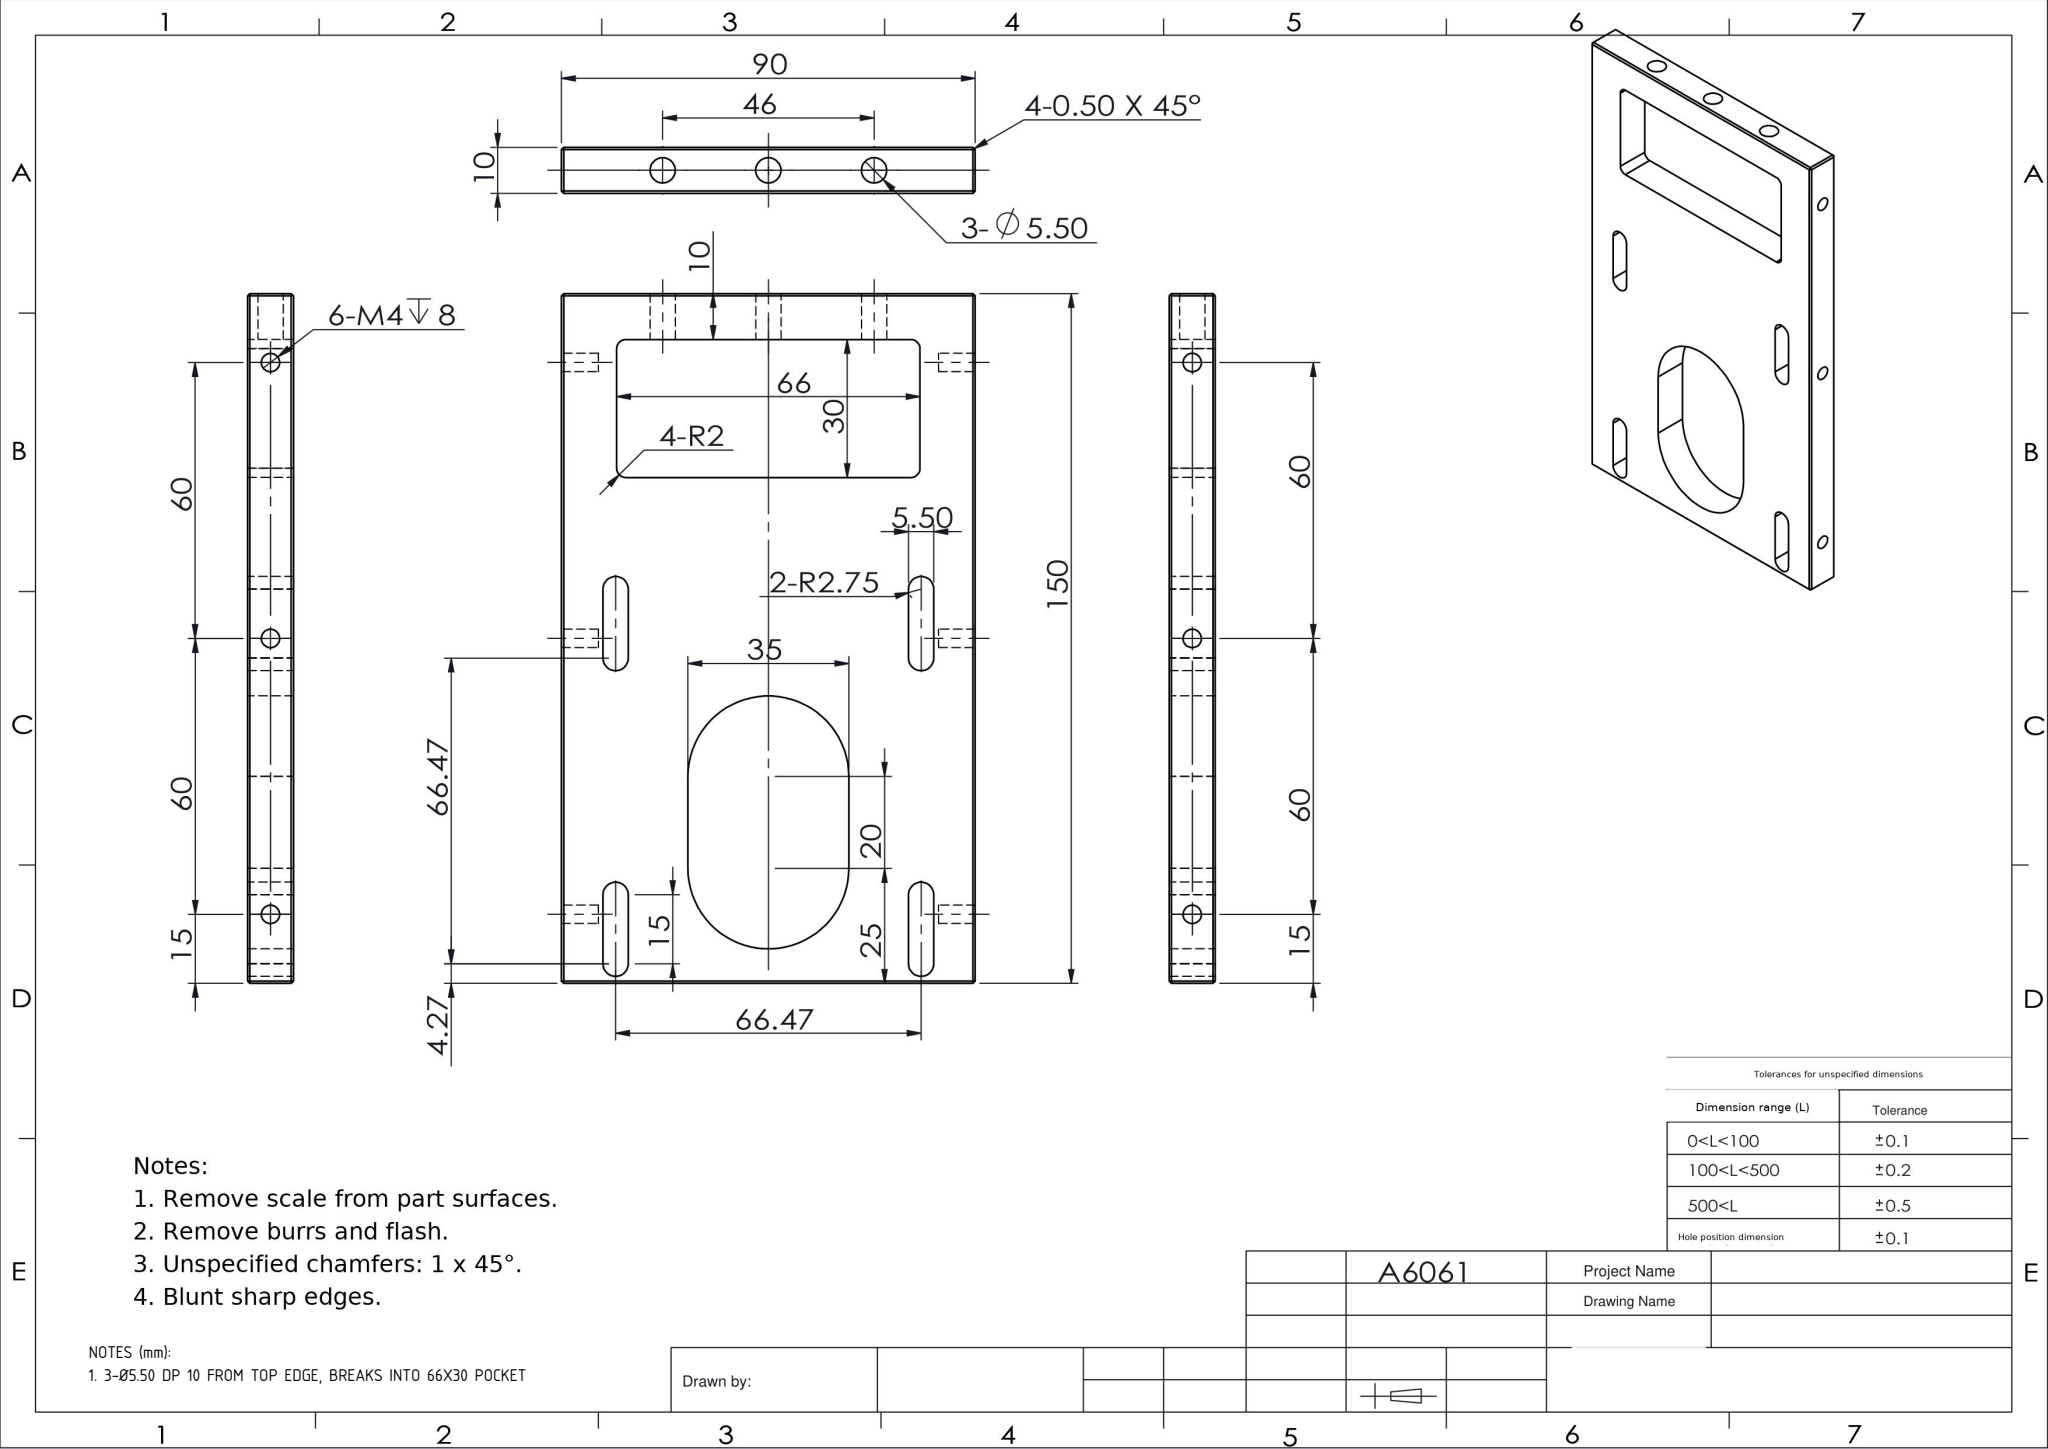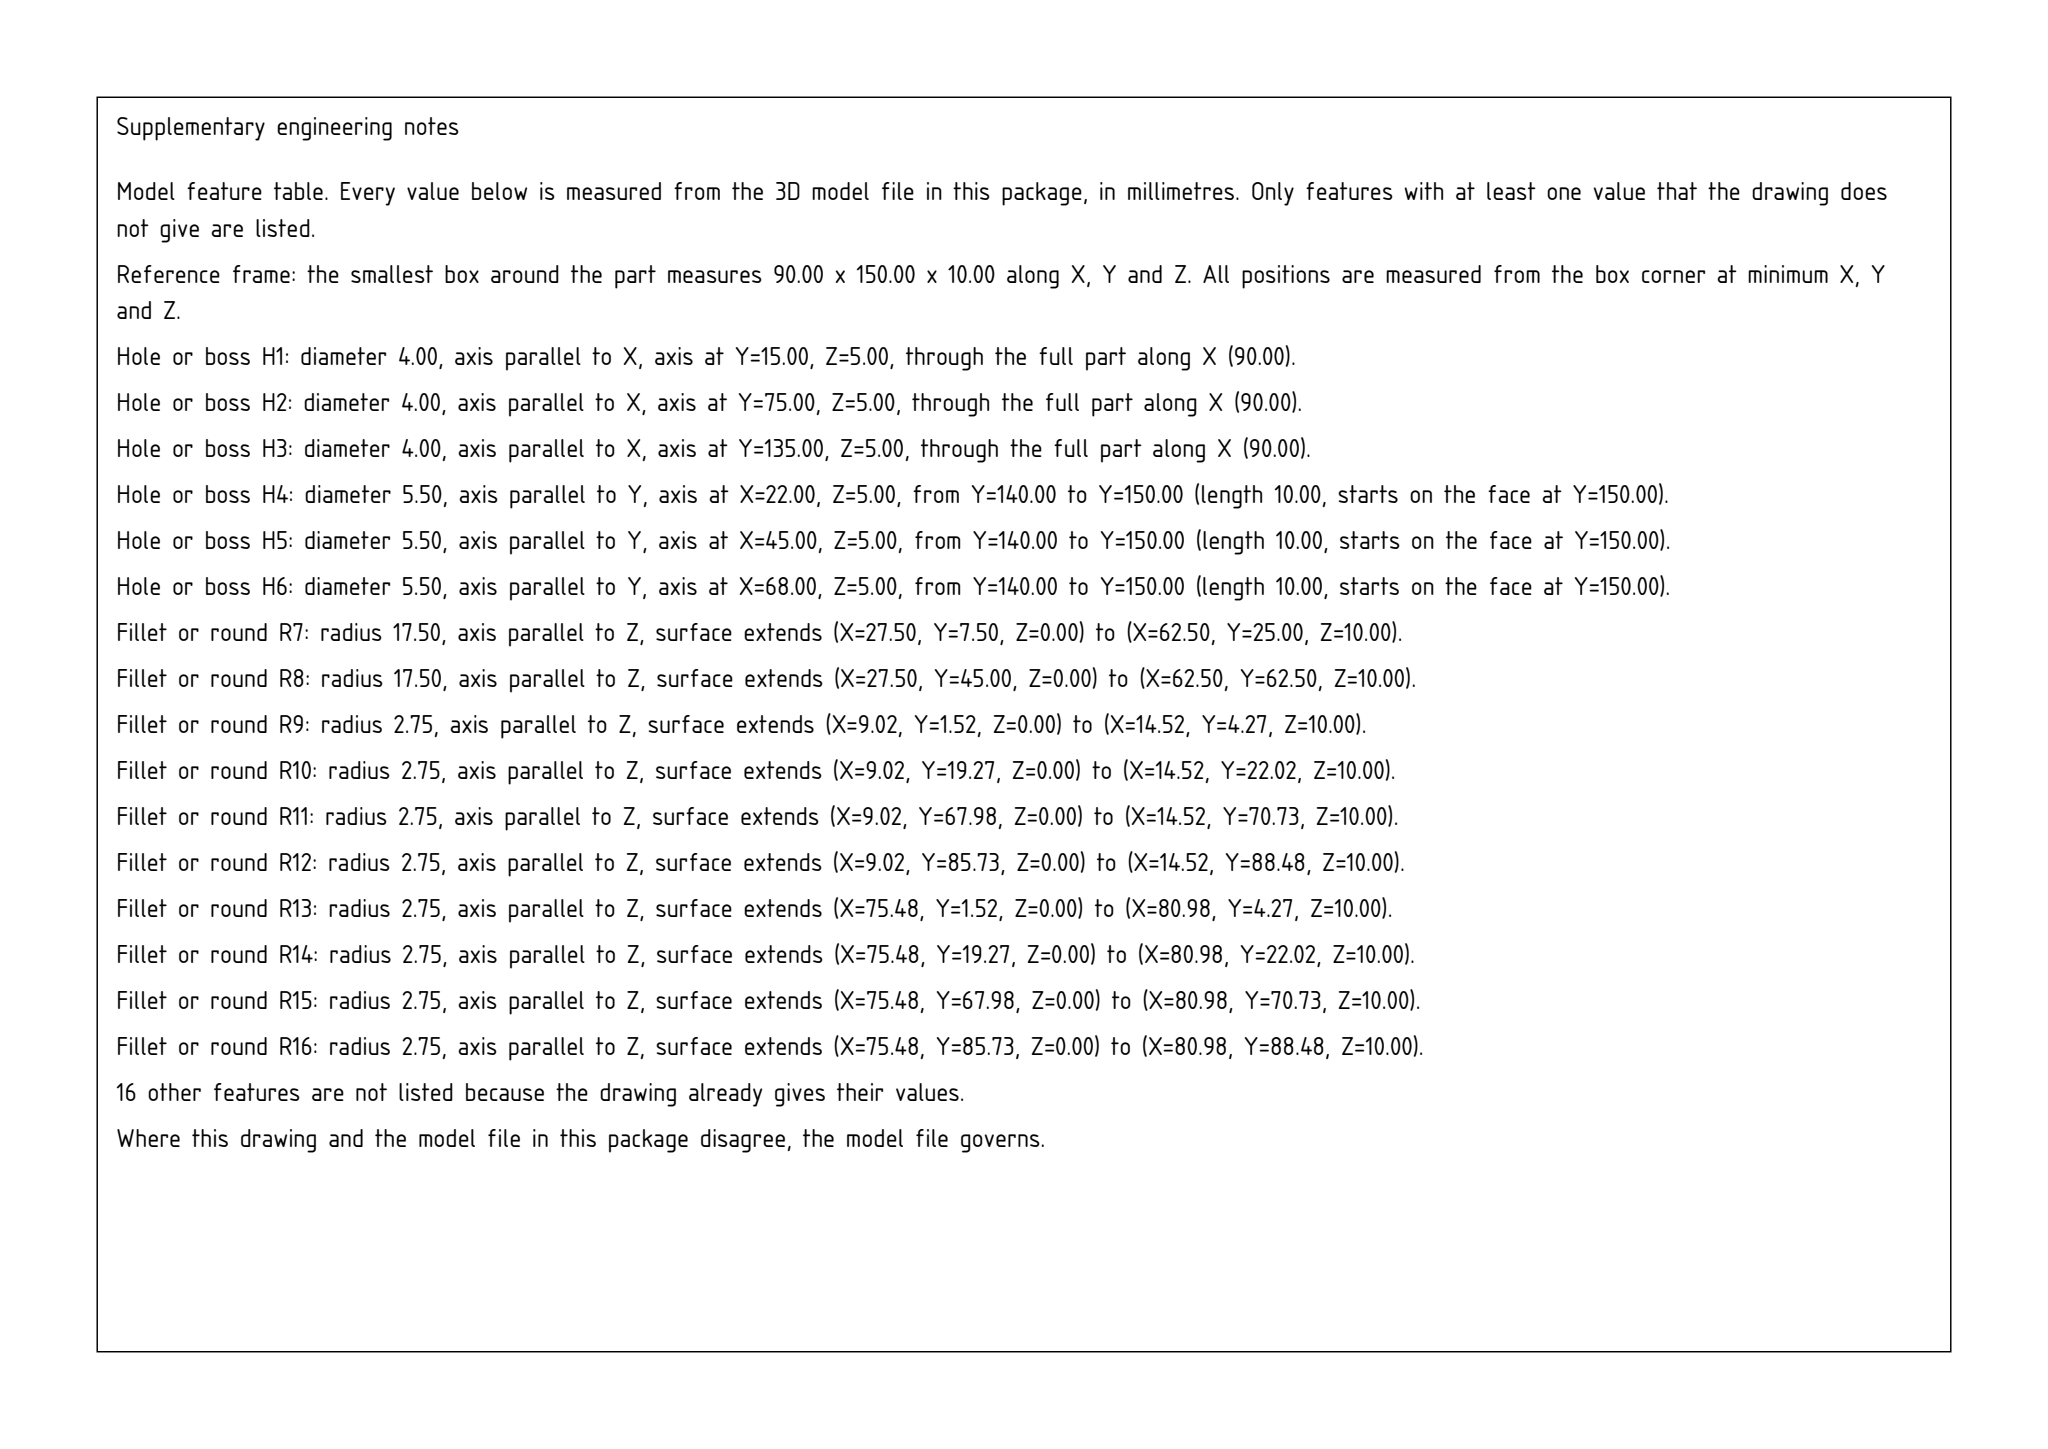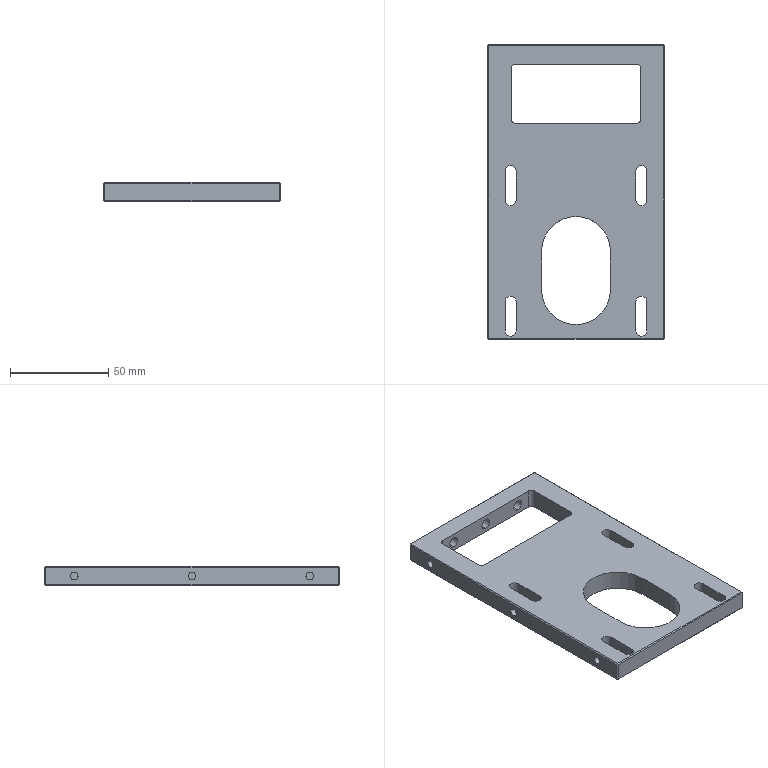Part | SolidWorks | mm | 1 solid | 78 faces | box 90 x 150 x 10 mm | volume 92923 mm3 | plane 46 | cylinder 32 | commonest cylinder face diameters 4 x16 5.5 x14 35 x2
Drawing notes:
3-Ø5.50 DP 10 FROM TOP EDGE, BREAKS INTO 66X30 POCKET | from the solid: Cyl dia5.5 axis y at x=22,45,68, z=5, len 10; from y=150 face to pocket face y=140
build123d program:
from build123d import *

# Parameters (mm, degrees)
SKETCH1_W           = 90
SKETCH1_H           = 150
BOSS_EXTRUDE1_DEPTH = 5
SKETCH5_R           = 2.1
CUT_EXTRUDE1_DEPTH  = 89.034
SKETCH6_R           = 17.5
CUT_EXTRUDE2_DEPTH  = 89.034
CHAMFER1_SIZE       = 0.5
CUT_EXTRUDE3_DEPTH  = 89.034
CUT_EXTRUDE4_DEPTH  = 89.034
SKETCH11_W          = 66
SKETCH11_H          = 30
CUT_EXTRUDE5_DEPTH  = 89.034
FILLET1_R           = 2
SKETCH13_R          = 2.75
CUT_EXTRUDE6_DEPTH  = 20
SKETCH14_R          = 2
CUT_EXTRUDE7_DEPTH  = 8
LPATTERN1_COUNT     = 3
LPATTERN1_PITCH     = 60
CUT_EXTRUDE8_START  = -8
SKETCH15_R          = 2
CUT_EXTRUDE8_DEPTH  = 8
LPATTERN2_COUNT     = 3
LPATTERN2_PITCH     = 60


with BuildPart() as part:
    # Sketch1 → Boss-Extrude1 (new, symmetric)
    with BuildSketch(Plane.XY):
        Rectangle(SKETCH1_W, SKETCH1_H)
    extrude(amount=BOSS_EXTRUDE1_DEPTH, both=True)

    # Sketch5 → Cut-Extrude1 (cut, through all)
    with BuildSketch(Plane(origin=(0, 0, -5), x_dir=(-1, 0, 0), z_dir=(0, 0, -1))):
        with Locations((-33.234, 3.234)):
            Circle(SKETCH5_R)
        with Locations((33.234, 3.234)):
            Circle(SKETCH5_R)
        with Locations((-33.234, -63.234)):
            Circle(SKETCH5_R)
        with Locations((33.234, -63.234)):
            Circle(SKETCH5_R)
    extrude(amount=-CUT_EXTRUDE1_DEPTH, mode=Mode.SUBTRACT)

    # Sketch6 → Cut-Extrude2 (cut, through all)
    with BuildSketch(Plane.XY.offset(5)):
        with Locations((0, -42)):
            Circle(SKETCH6_R)
    extrude(amount=-CUT_EXTRUDE2_DEPTH, mode=Mode.SUBTRACT)

    # Chamfer1
    chamfer1_edges = [part.edges().sort_by_distance(p)[0] for p in [
        (-45, 0, 5),
        (0, -75, 5),
        (45, 0, 5),
        (0, -75, -5),
        (-45, 0, -5),
        (0, 75, -5),
        (45, 0, -5),
        (0, 75, 5),
        (45, -75, 0),
        (-45, -75, 0),
        (-45, 75, 0),
        (45, 75, 0),
    ]]
    chamfer(chamfer1_edges, length=CHAMFER1_SIZE)

    # Sketch9 → Cut-Extrude3 (cut, through all)
    with BuildSketch(Plane.XY.offset(5)):
        with BuildLine():
            Line((-30.484, 10.734), (-30.484, -4.266))
            ThreePointArc((-30.484, -4.266), (-33.234, -7.016), (-35.984, -4.266))
            Line((-35.984, -4.266), (-35.984, 10.734))
            ThreePointArc((-35.984, 10.734), (-33.234, 13.484), (-30.484, 10.734))
        make_face()
        with BuildLine():
            Line((35.984, 10.734), (35.984, -4.266))
            ThreePointArc((35.984, -4.266), (33.234, -7.016), (30.484, -4.266))
            Line((30.484, -4.266), (30.484, 10.734))
            ThreePointArc((30.484, 10.734), (33.234, 13.484), (35.984, 10.734))
        make_face()
        with BuildLine():
            Line((-30.484, -55.734), (-30.484, -70.734))
            ThreePointArc((-30.484, -70.734), (-33.234, -73.484), (-35.984, -70.734))
            Line((-35.984, -70.734), (-35.984, -55.734))
            ThreePointArc((-35.984, -55.734), (-33.234, -52.984), (-30.484, -55.734))
        make_face()
        with BuildLine():
            Line((35.984, -55.734), (35.984, -70.734))
            ThreePointArc((35.984, -70.734), (33.234, -73.484), (30.484, -70.734))
            Line((30.484, -70.734), (30.484, -55.734))
            ThreePointArc((30.484, -55.734), (33.234, -52.984), (35.984, -55.734))
        make_face()
    extrude(amount=-CUT_EXTRUDE3_DEPTH, mode=Mode.SUBTRACT)

    # Sketch10 → Cut-Extrude4 (cut, through all)
    with BuildSketch(Plane.XY.offset(5)):
        with BuildLine():
            Line((17.5, -30), (17.5, -50))
            ThreePointArc((17.5, -50), (0, -67.5), (-17.5, -50))
            Line((-17.5, -50), (-17.5, -30))
            ThreePointArc((-17.5, -30), (0, -12.5), (17.5, -30))
        make_face()
    extrude(amount=-CUT_EXTRUDE4_DEPTH, mode=Mode.SUBTRACT)

    # Sketch11 → Cut-Extrude5 (cut, through all)
    with BuildSketch(Plane(origin=(0, 0, -5), x_dir=(-1, 0, 0), z_dir=(0, 0, -1))):
        with Locations((0, 50)):
            Rectangle(SKETCH11_W, SKETCH11_H)
    extrude(amount=-CUT_EXTRUDE5_DEPTH, mode=Mode.SUBTRACT)

    # Fillet1
    fillet1_edges = [part.edges().sort_by_distance(p)[0] for p in [
        (33, 35, 0),
        (33, 65, 0),
        (-33, 65, 0),
        (-33, 35, 0),
    ]]
    fillet(fillet1_edges, radius=FILLET1_R)

    # Sketch13 → Cut-Extrude6 (cut)
    with BuildSketch(Plane(origin=(0, 75, 0), x_dir=(1, 0, 0), z_dir=(0, 1, 0))):
        with Locations(Location((-23, 0, 0), (0, 0, 270))):
            Circle(SKETCH13_R)
        with Locations(Location((0, 0, 0), (0, 0, 270))):
            Circle(SKETCH13_R)
        with Locations(Location((23, 0, 0), (0, 0, 270))):
            Circle(SKETCH13_R)
    extrude(amount=-CUT_EXTRUDE6_DEPTH, mode=Mode.SUBTRACT)

    # Sketch14 → Cut-Extrude7 (cut)
    with BuildSketch(Plane(origin=(45, 0, 0), x_dir=(0, 0, -1), z_dir=(1, 0, 0))):
        with Locations(Location((0, 60, 0), (0, 0, 90))):
            Circle(SKETCH14_R)
    cut_extrude7 = extrude(amount=-CUT_EXTRUDE7_DEPTH, mode=Mode.SUBTRACT)

    # LPattern1: Cut-Extrude7 ×3
    with Locations(*[(0, -i * LPATTERN1_PITCH, 0) for i in range(1, LPATTERN1_COUNT)]):
        add(cut_extrude7, mode=Mode.SUBTRACT)

    # Sketch15 → Cut-Extrude8 (cut)
    with BuildSketch(Plane.ZY.offset(45).offset(CUT_EXTRUDE8_START)):
        with Locations(Location((0, 60, 0), (0, 0, 90))):
            Circle(SKETCH15_R)
    cut_extrude8 = extrude(amount=CUT_EXTRUDE8_DEPTH, mode=Mode.SUBTRACT)

    # LPattern2: Cut-Extrude8 ×3
    with Locations(*[(0, -i * LPATTERN2_PITCH, 0) for i in range(1, LPATTERN2_COUNT)]):
        add(cut_extrude8, mode=Mode.SUBTRACT)


solid = part.part